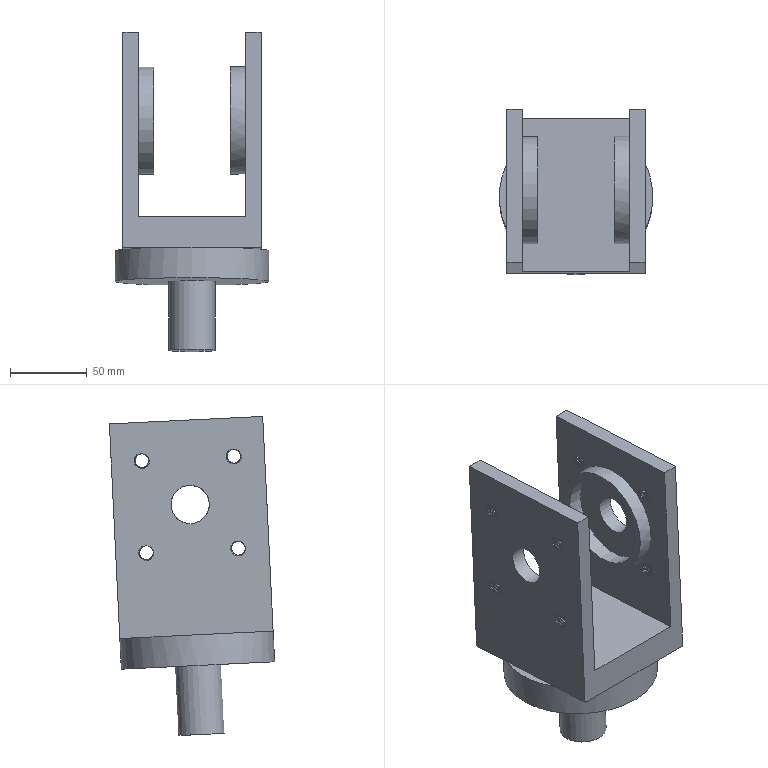Component | NX | CCJ-008 | 1 solid | 83 faces | volume 613720 mm3 | cylinder 36 | plane 31 | spline 16 | commonest cylinder face diameters 10 x20 9 x8 70 x2 60 x2 25 x2 100 x1 30 x1